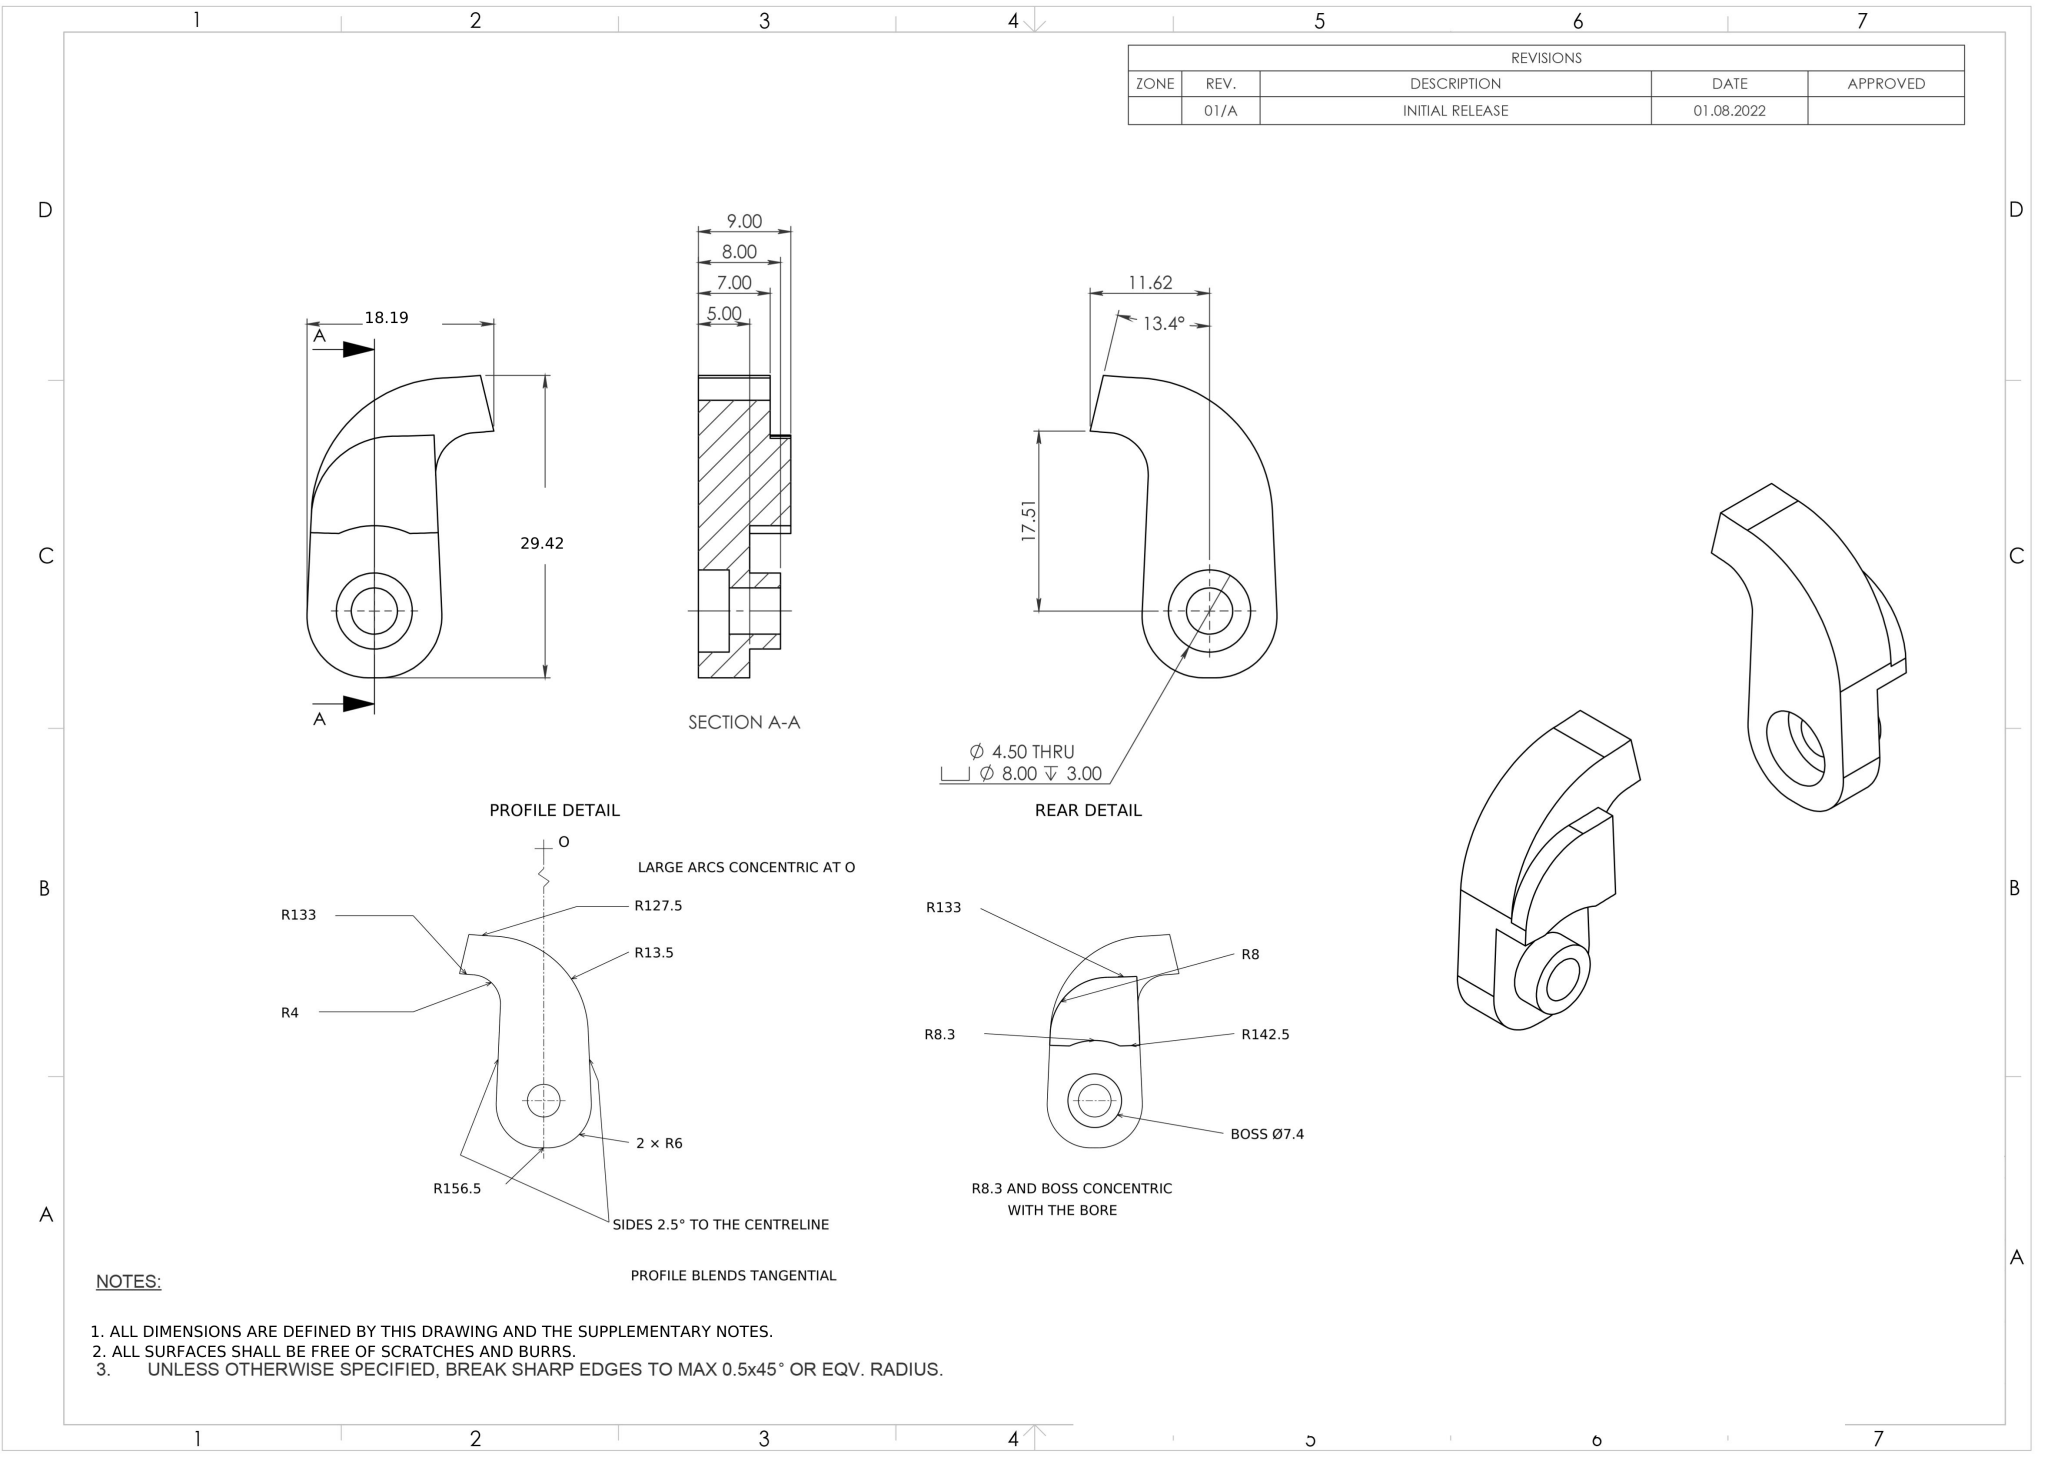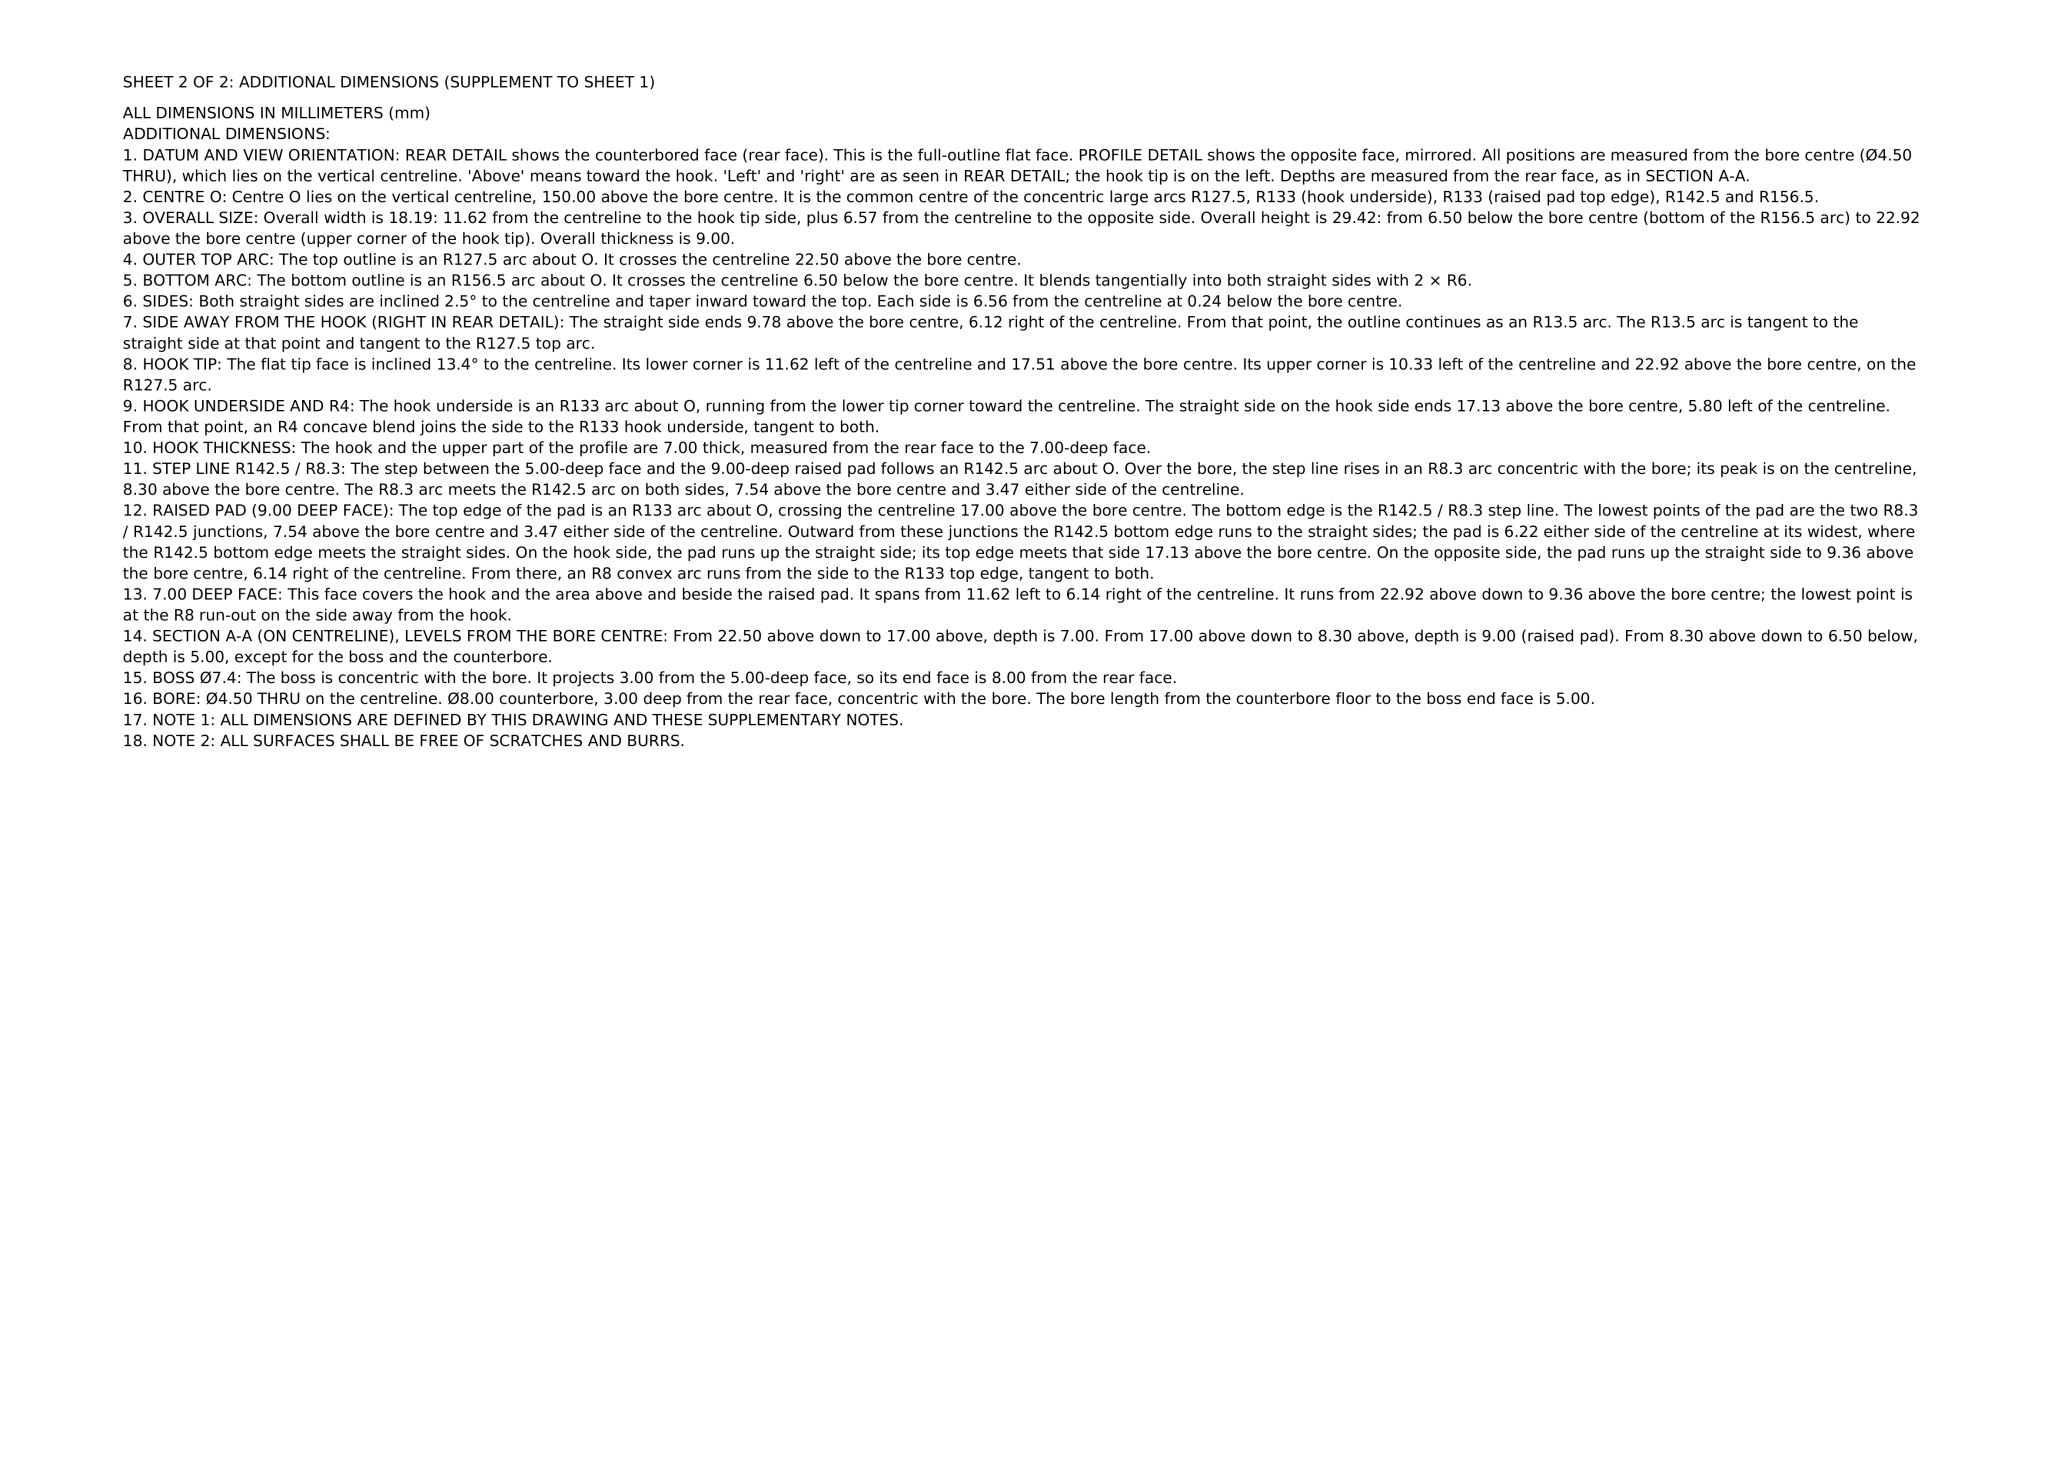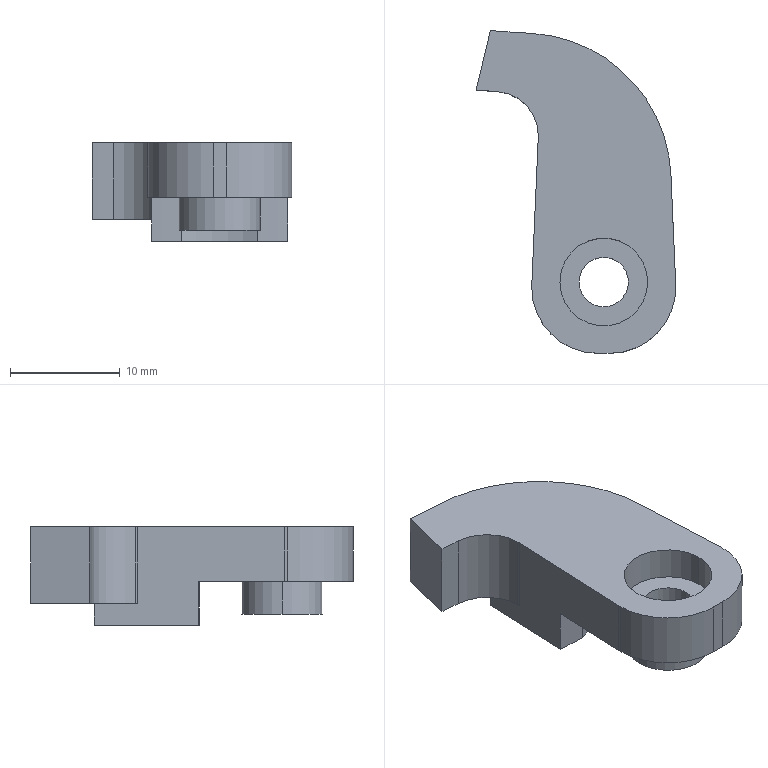Part | NX | mm | 1 solid | 29 faces | box 18.19 x 29.42 x 9 mm | volume 2148 mm3 | cylinder 20 | plane 9 | commonest cylinder face diameters 8 x4 12 x3 7.4 x2 4.5 x2 285 x2 266 x2 255 x1 313 x1